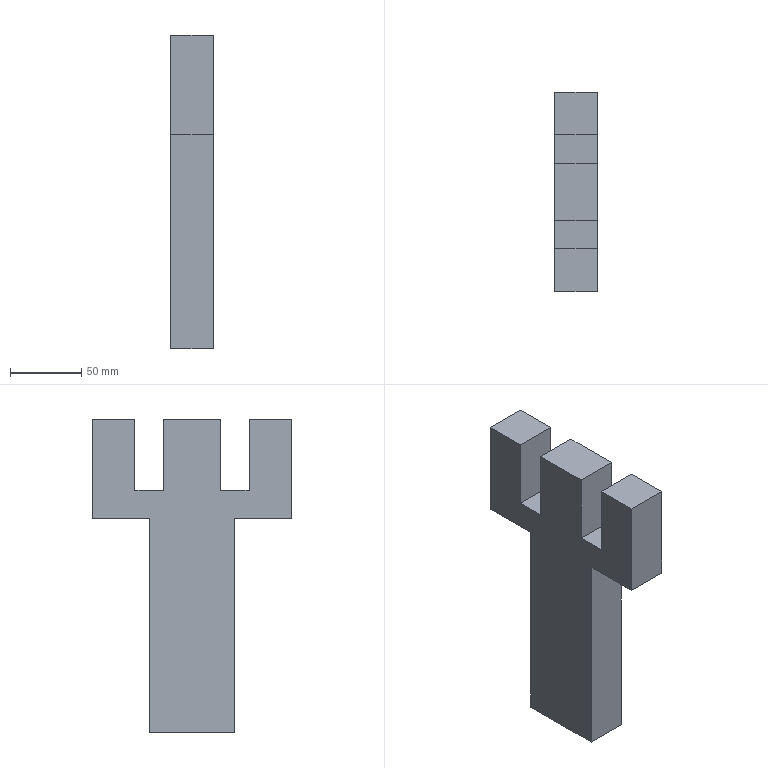Component | NX | CATAL_2 | 1 solid | 18 faces | volume 504000 mm3 | plane 18